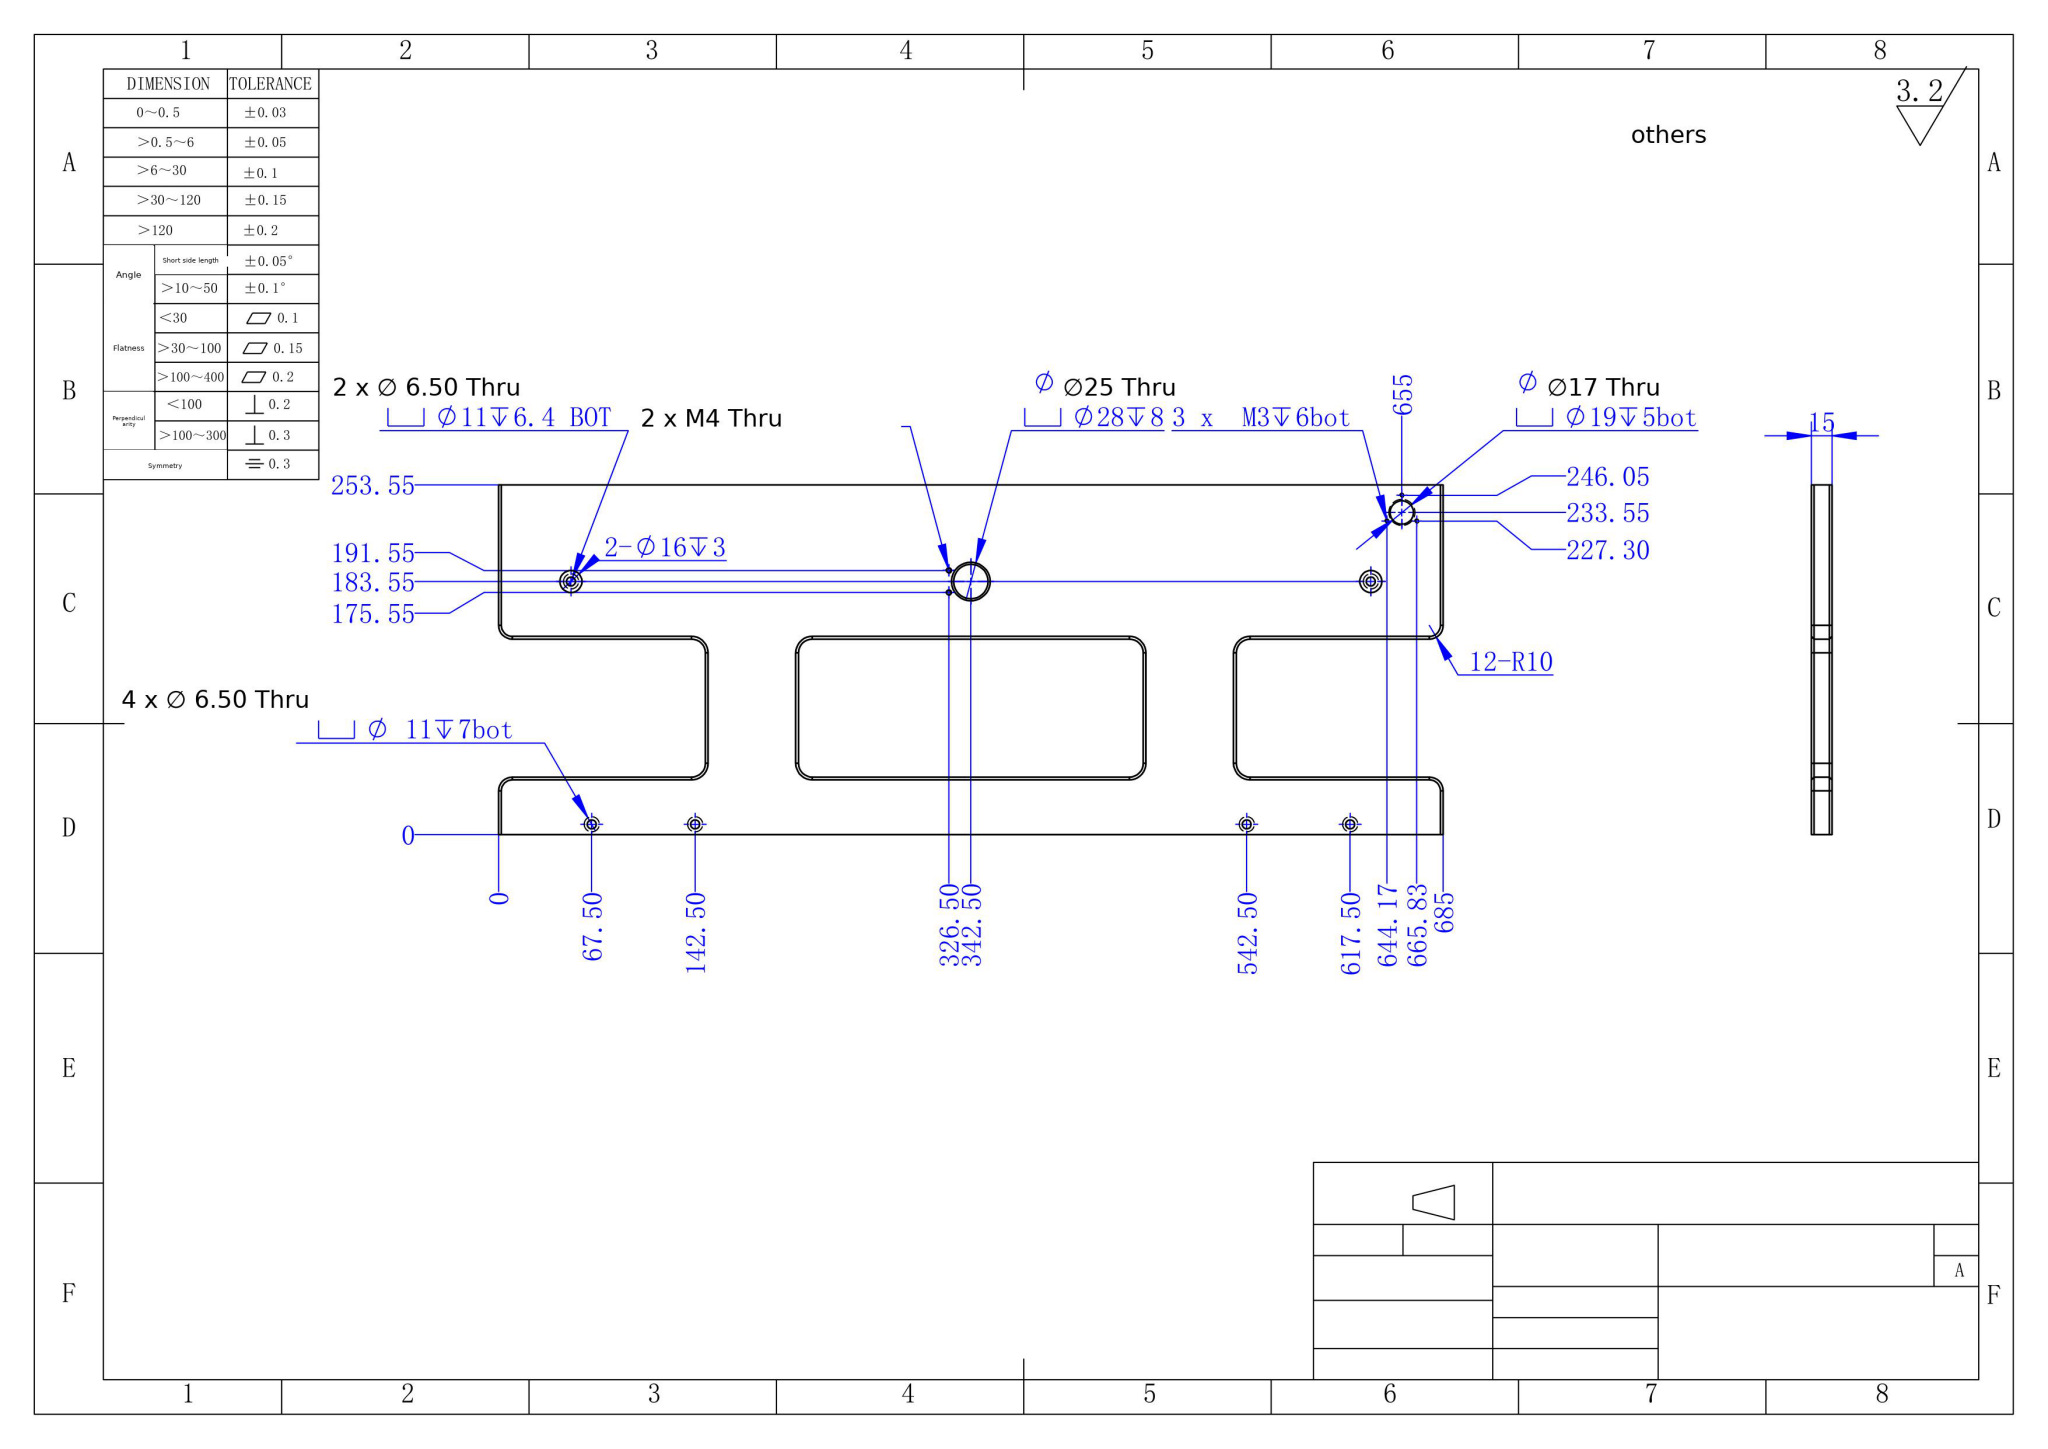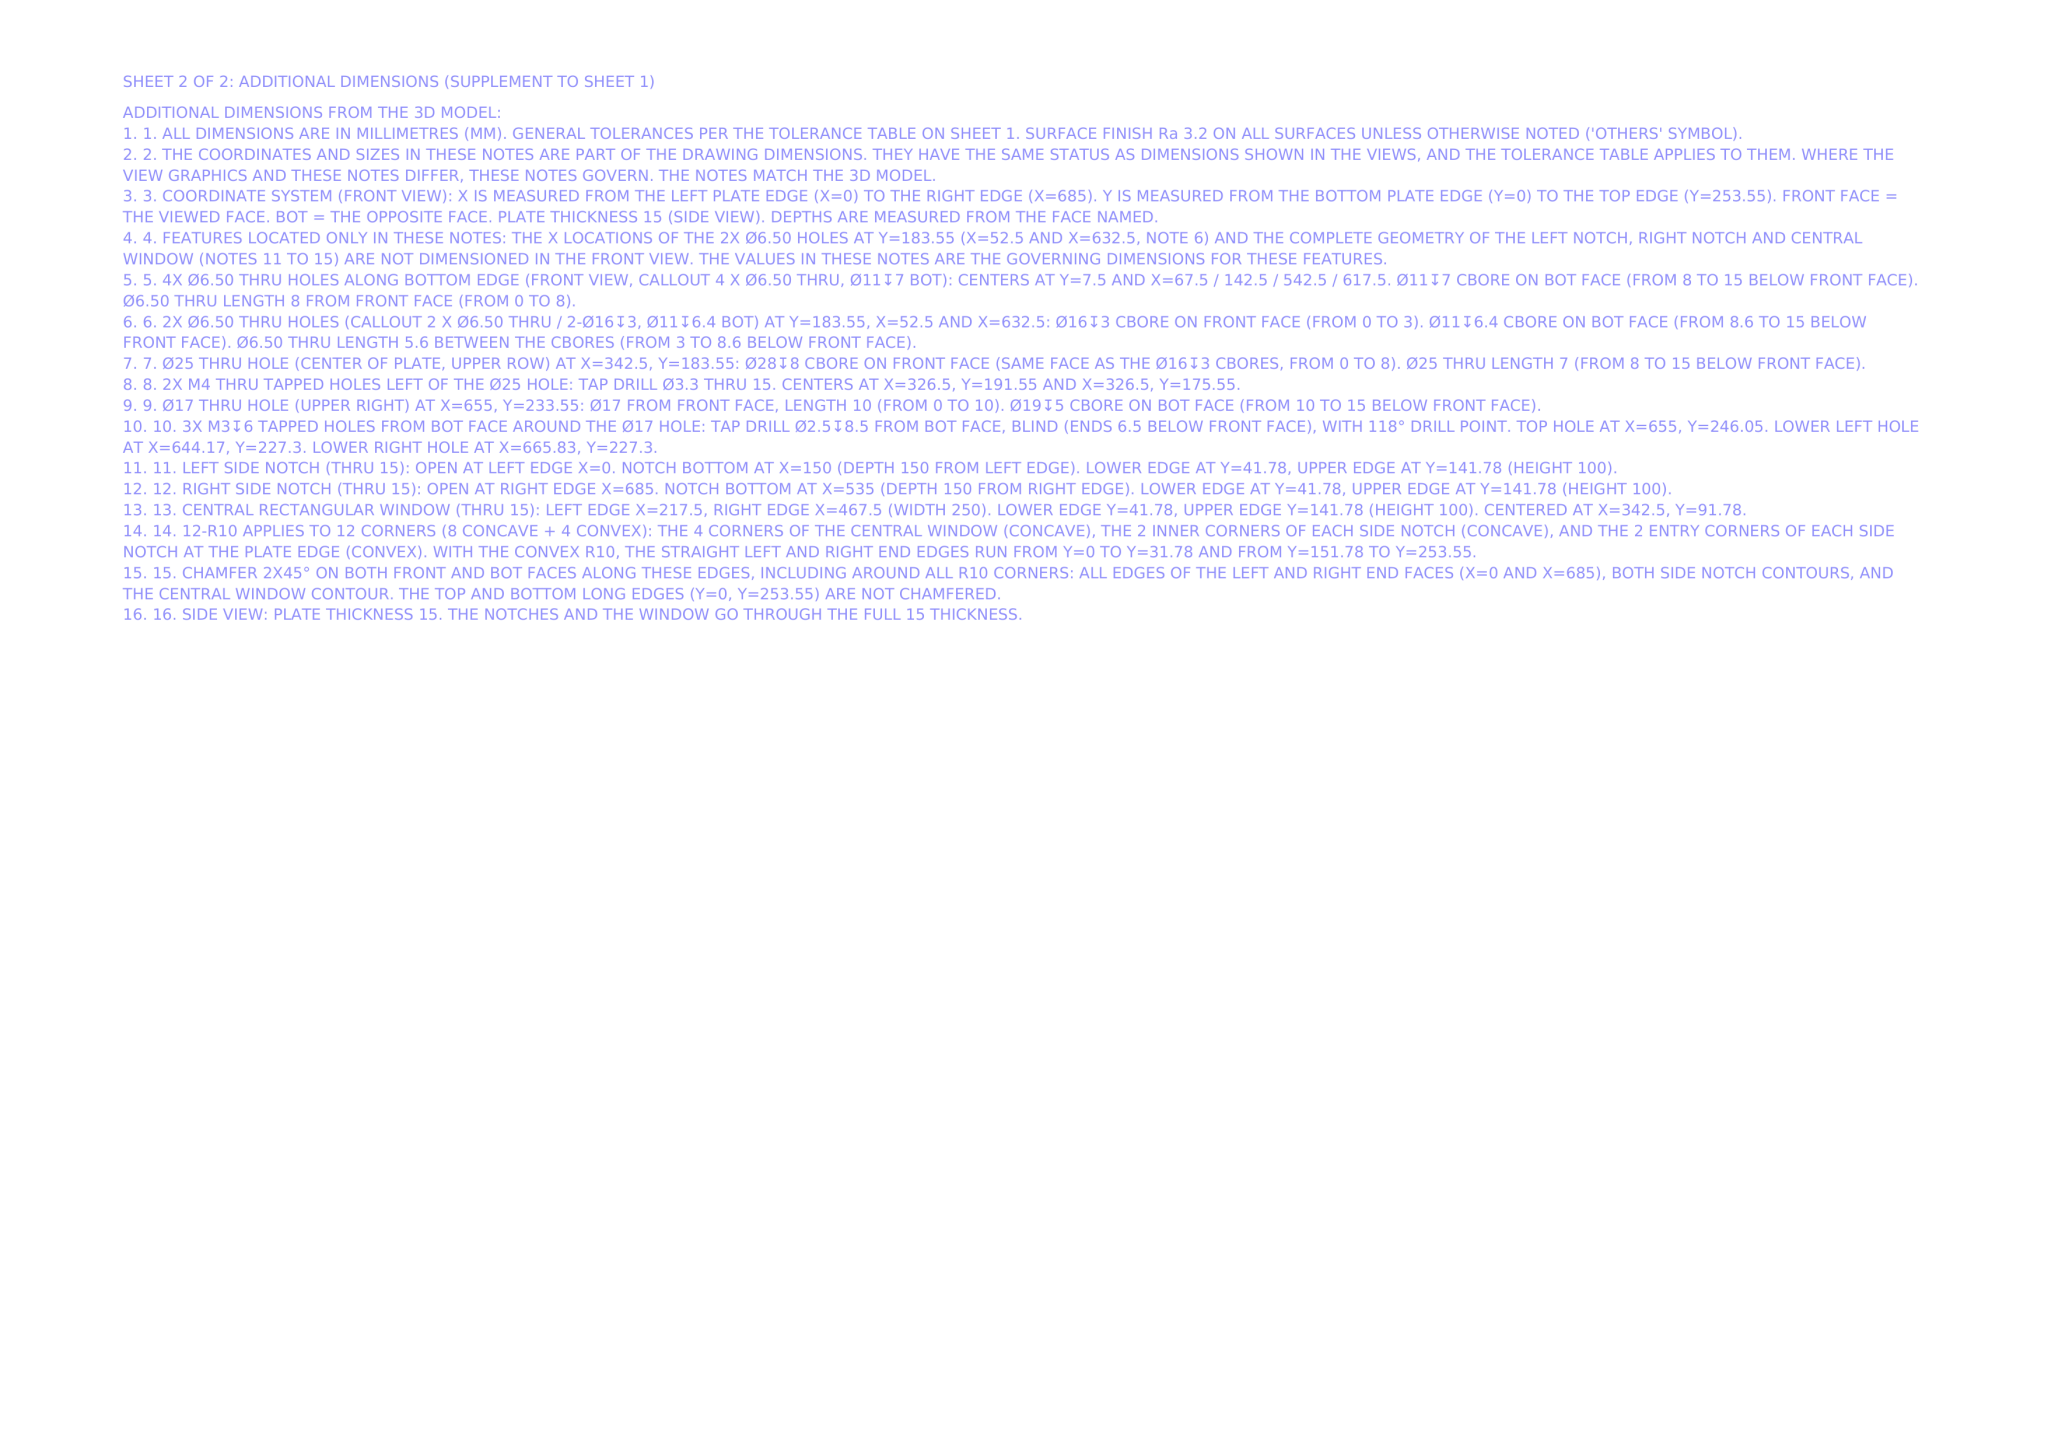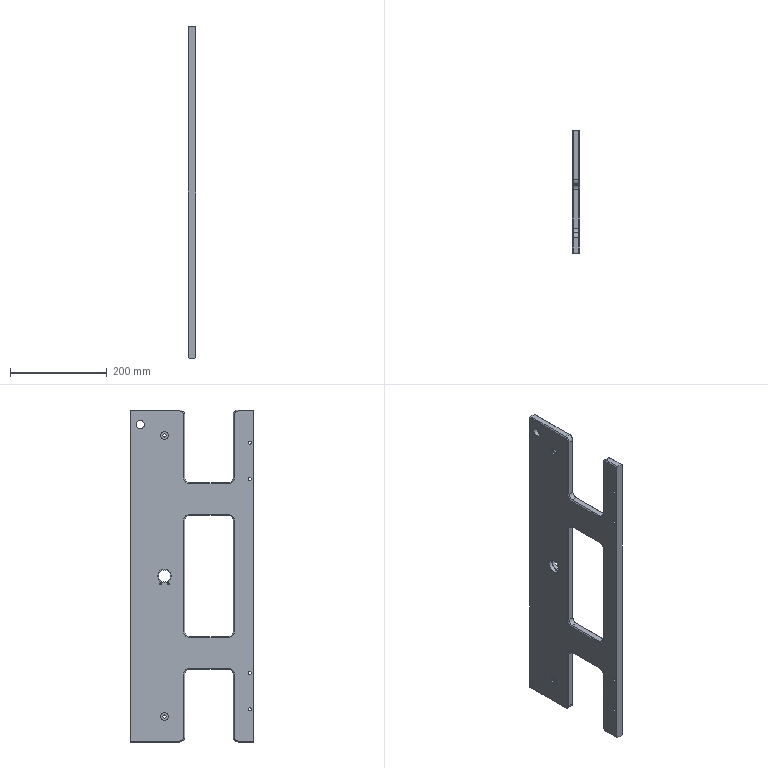Part | NX | mm | 1 solid | 144 faces | box 15 x 253.55 x 685 mm | volume 1755522 mm3 | cylinder 58 | plane 56 | cone 30 | commonest cylinder face diameters 11 x12 6.5 x12 20 x12 2.5 x6 3.3 x4 16 x4 25 x2 28 x2